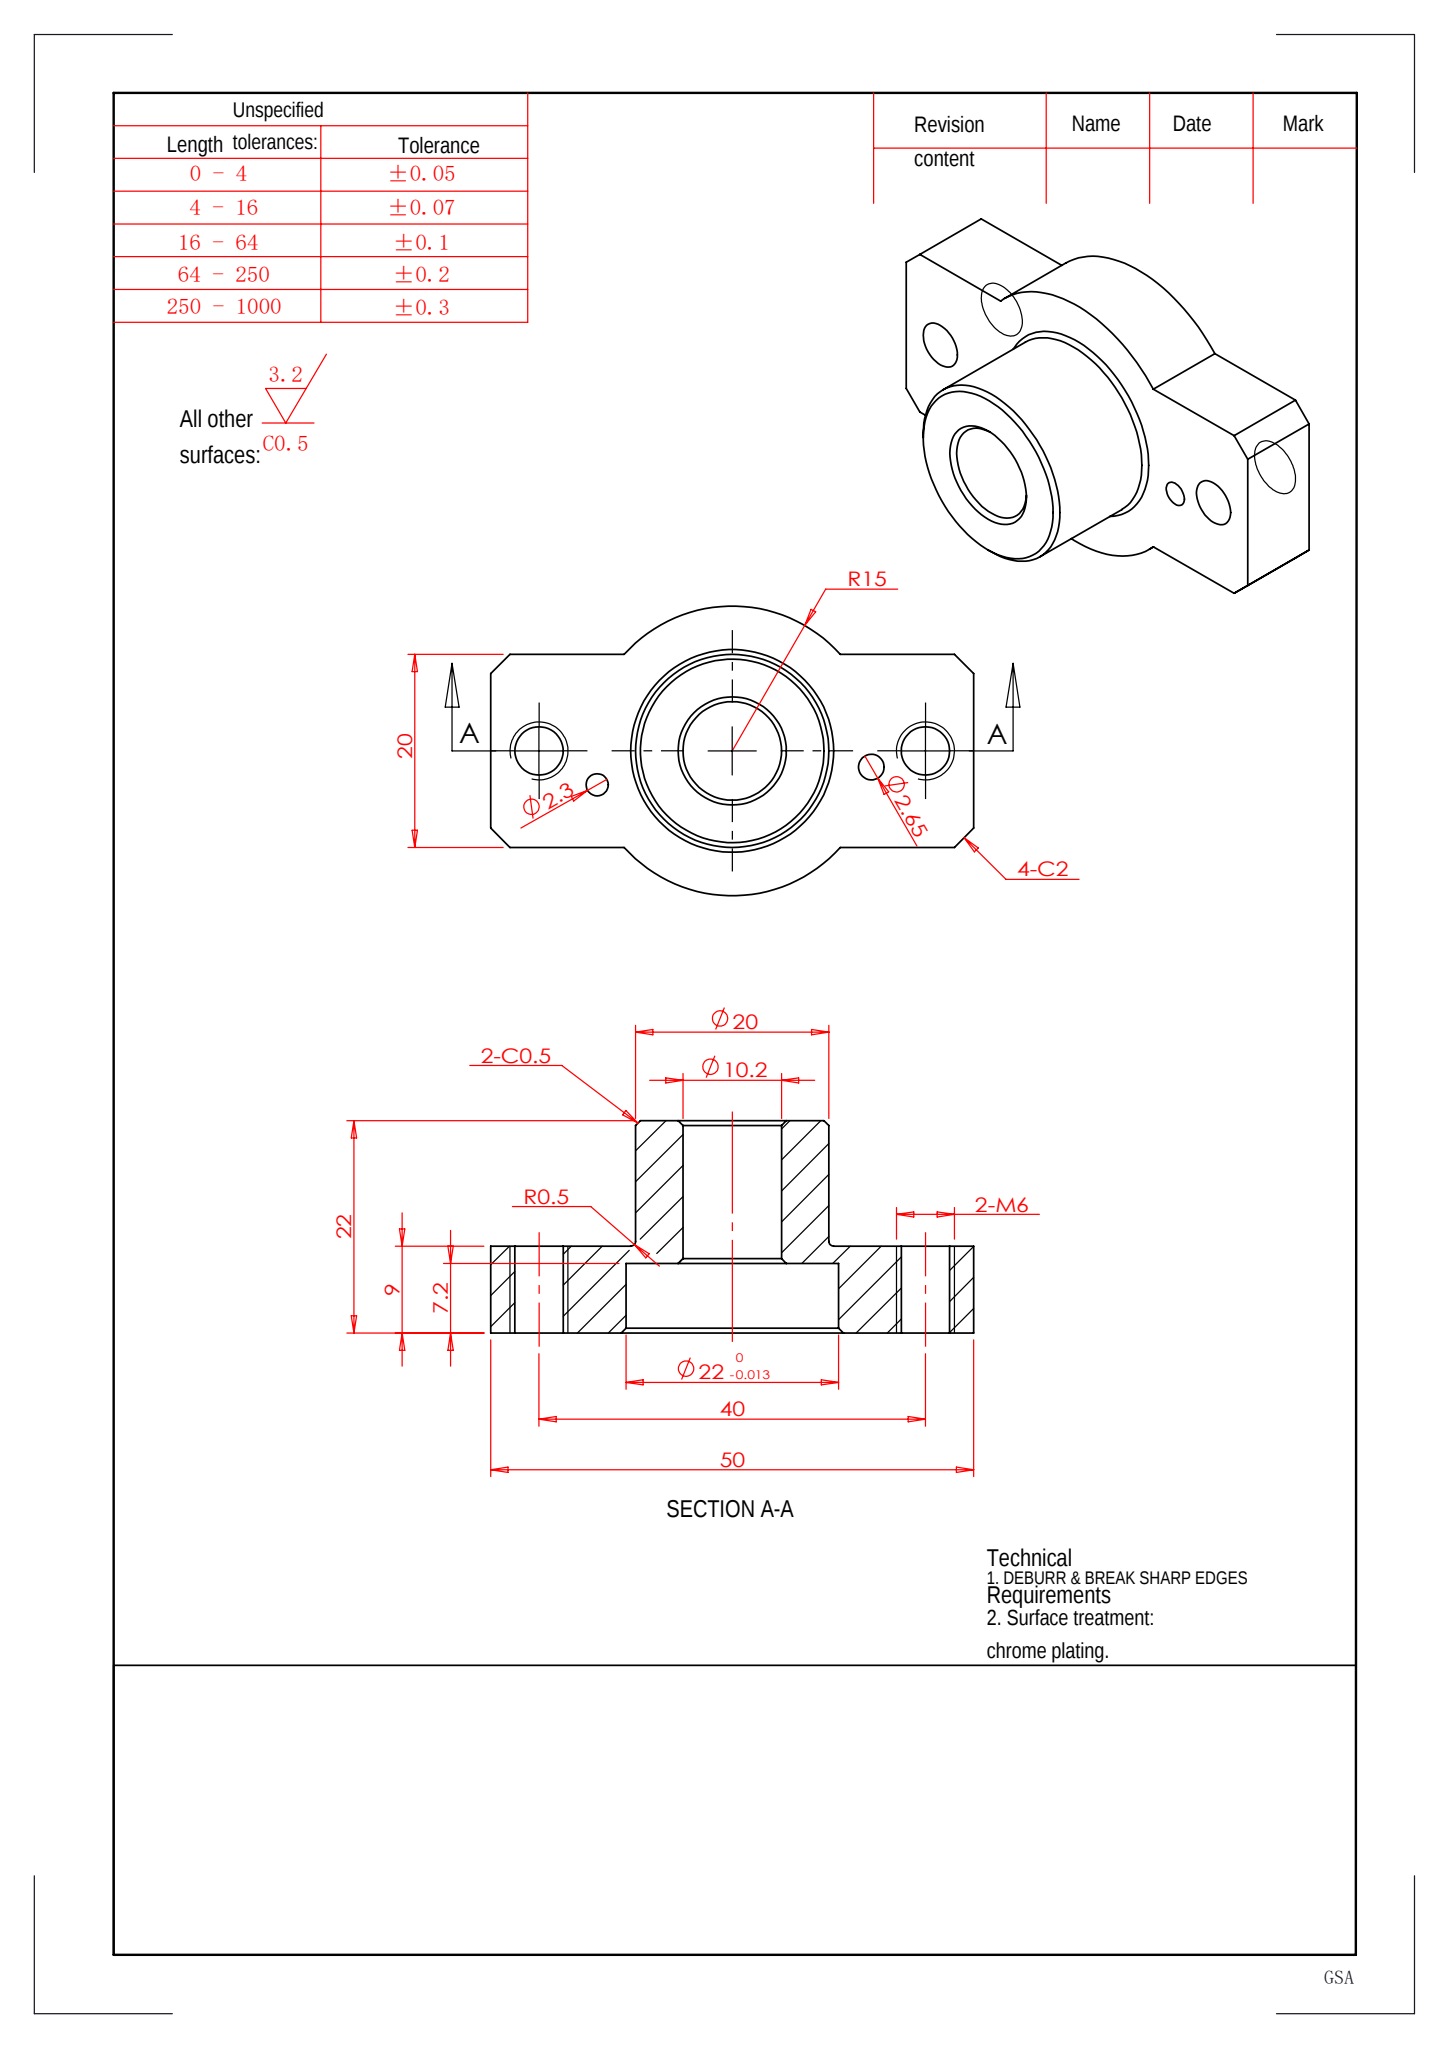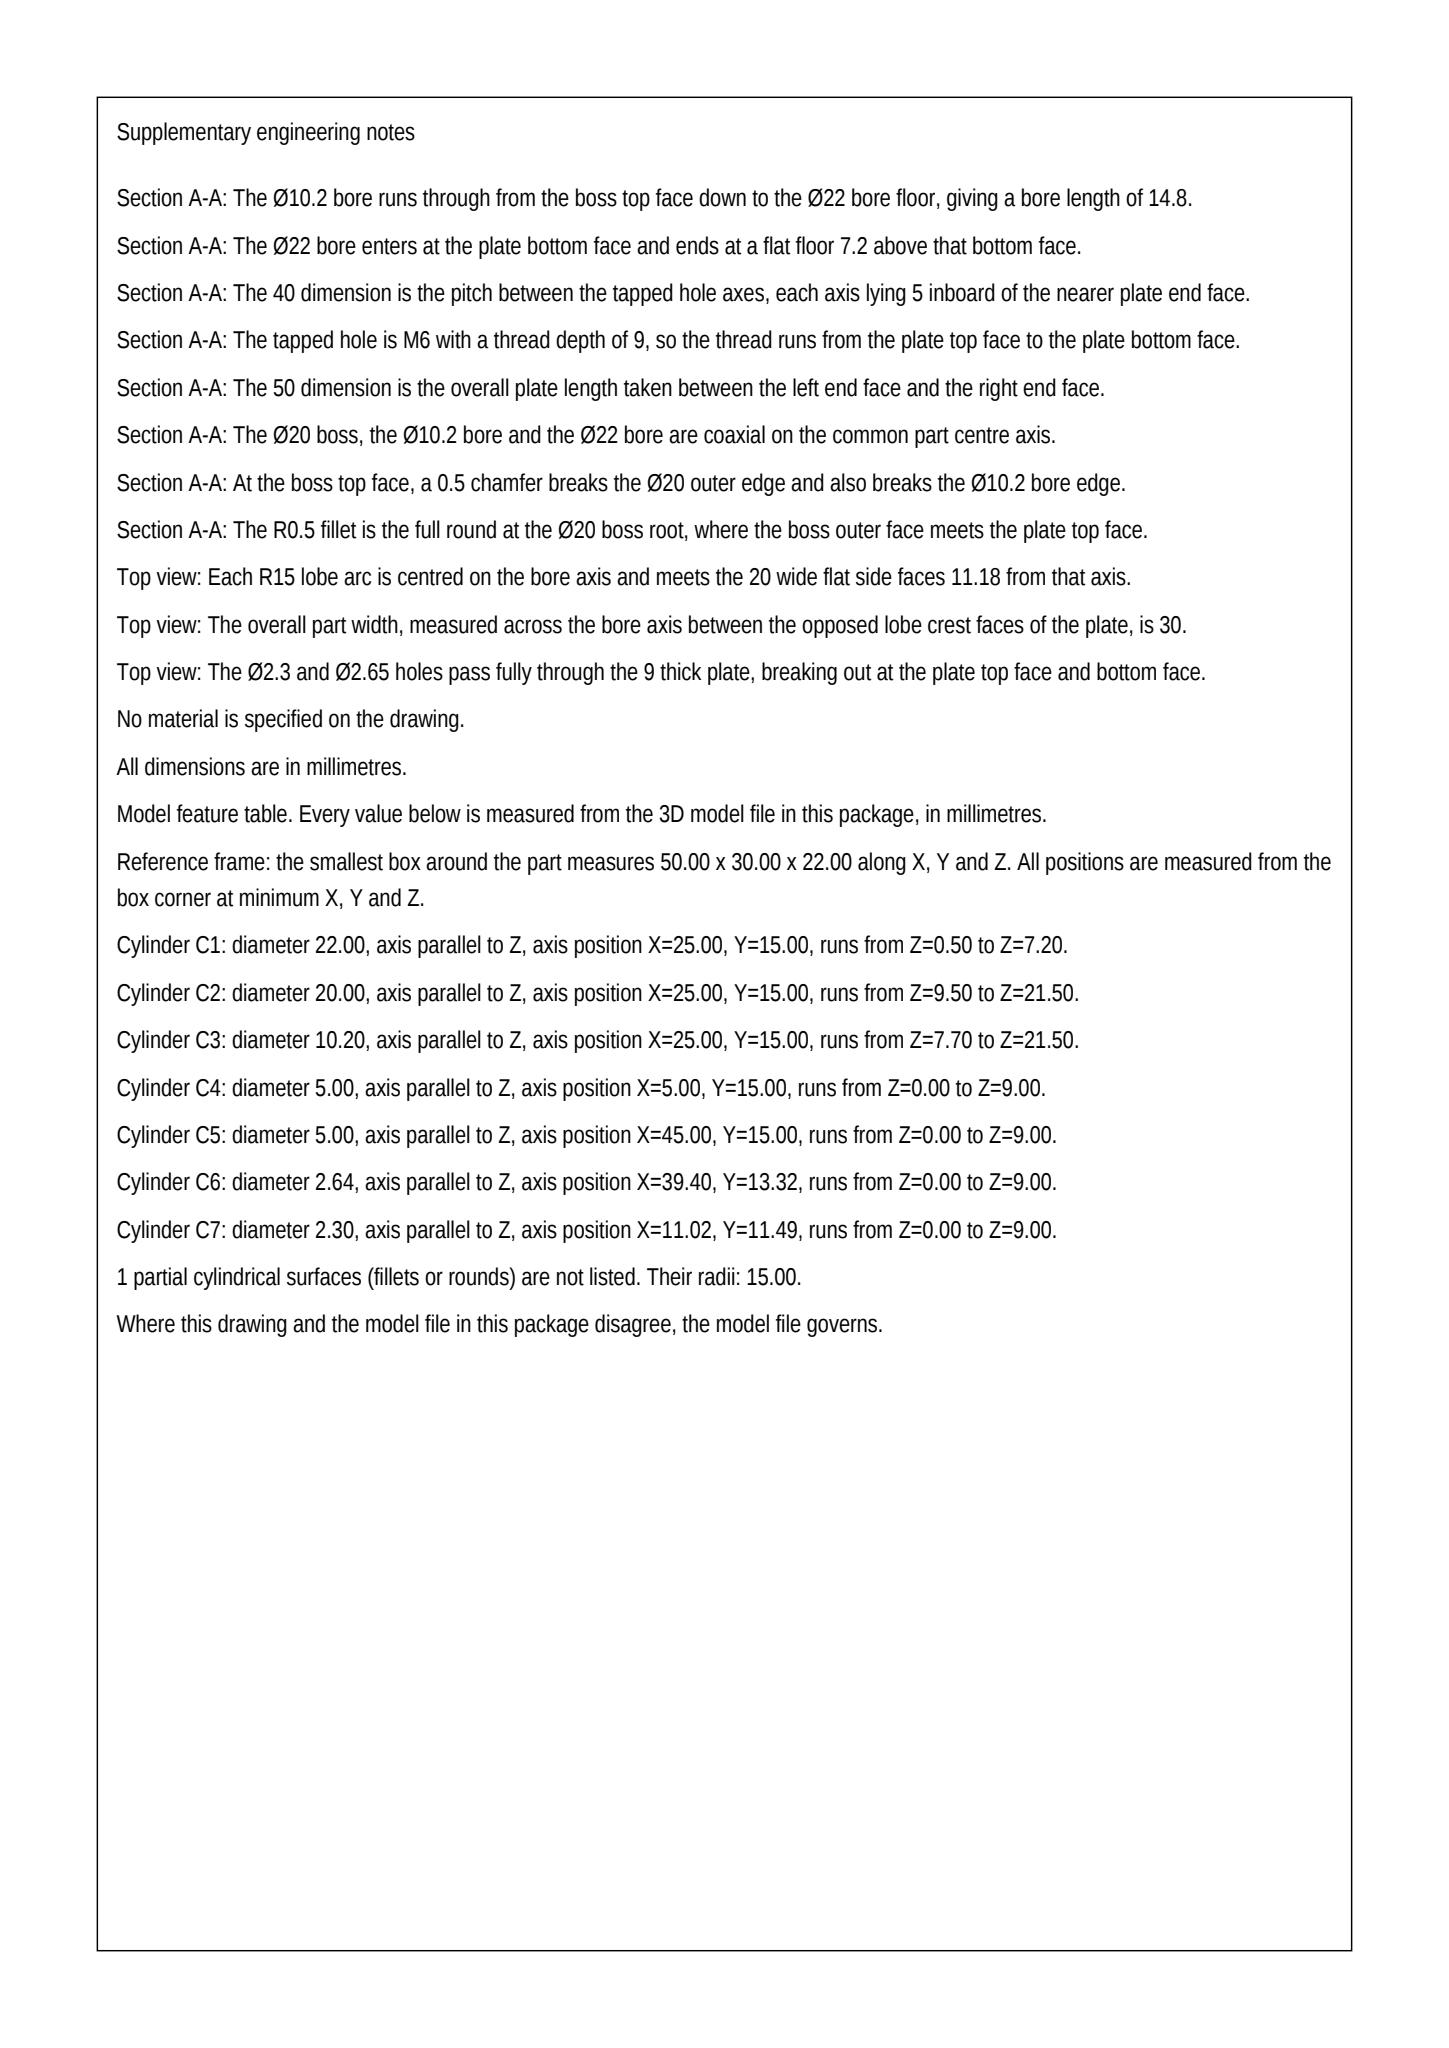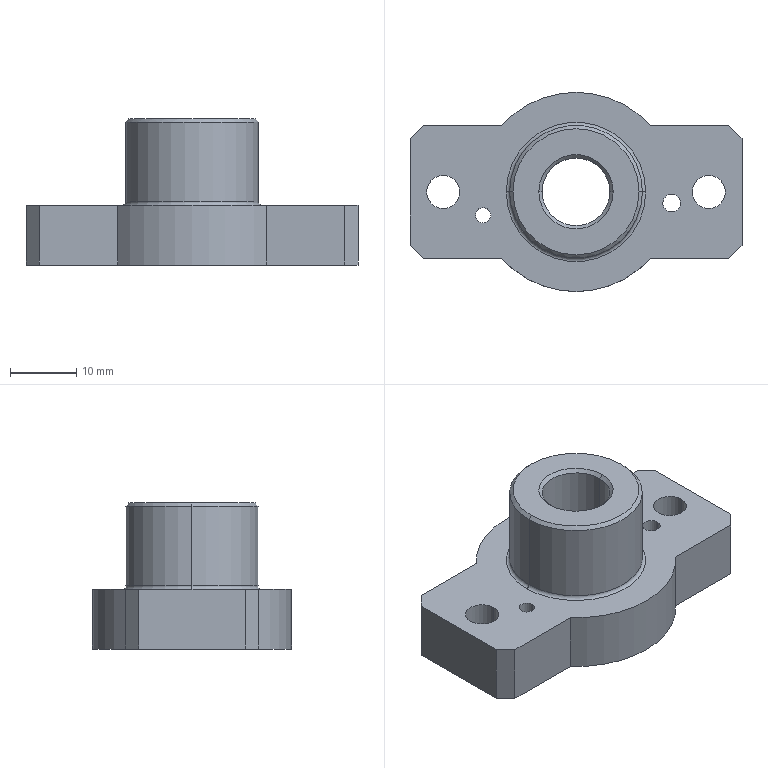Part | SolidWorks | mm | 1 solid | 40 faces | box 50 x 30 x 22 mm | volume 9998 mm3 | cylinder 16 | plane 14 | cone 8 | torus 2 | commonest cylinder face diameters 5 x4 2.65 x2 2.297 x2 22 x2 10.2 x2 20 x2 30 x2
build123d program:
from build123d import *

# Parameters (mm, degrees)
SKETCH1_R           = 1.5
BOSS_EXTRUDE1_DEPTH = 9
SKETCH2_R           = 10
SKETCH2_R_2         = 5.1
BOSS_EXTRUDE2_DEPTH = 13
SKETCH3_R           = 11
CUT_EXTRUDE1_DEPTH  = 7.2
SKETCH4_R           = 5.1
CUT_EXTRUDE2_DEPTH  = 32.922
CHAMFER1_SIZE       = 2
CHAMFER2_SIZE       = 0.5
FILLET1_R           = 0.5
M6_TAPPED_HOLE1_D   = 5
SKETCH7_R           = 1.325
SKETCH7_R_2         = 1.149
CUT_EXTRUDE3_DEPTH  = 27


with BuildPart() as part:
    # Sketch1 → Boss-Extrude1 (new body)
    with BuildSketch(Plane.XY):
        with BuildLine():
            Line((-25, -10), (-11.18, -10))
            ThreePointArc((-11.18, -10), (0, -15), (11.18, -10))
            Line((11.18, -10), (25, -10))
            Line((25, -10), (25, 10))
            Line((25, 10), (11.18, 10))
            ThreePointArc((11.18, 10), (0, 15), (-11.18, 10))
            Line((-11.18, 10), (-25, 10))
            Line((-25, 10), (-25, -10))
        make_face()
        with Locations((-20, 0)):
            Circle(SKETCH1_R, mode=Mode.SUBTRACT)
        with Locations((20, 0)):
            Circle(SKETCH1_R, mode=Mode.SUBTRACT)
    extrude(amount=BOSS_EXTRUDE1_DEPTH)

    # Sketch2 → Boss-Extrude2 (add)
    with BuildSketch(Plane.XY.offset(9)):
        with Locations(Location((0, 0, 0), (0, 0, 180))):
            Circle(SKETCH2_R)
        with Locations(Location((0, 0, 0), (0, 0, 180))):
            Circle(SKETCH2_R_2, mode=Mode.SUBTRACT)
    extrude(amount=BOSS_EXTRUDE2_DEPTH)

    # Sketch3 → Cut-Extrude1 (cut)
    with BuildSketch(Plane(origin=(0, 0, 0), x_dir=(-1, 0, 0), z_dir=(0, 0, -1))):
        Circle(SKETCH3_R)
    extrude(amount=-CUT_EXTRUDE1_DEPTH, mode=Mode.SUBTRACT)

    # Sketch4 → Cut-Extrude2 (cut, through all)
    with BuildSketch(Plane.XY.offset(9)):
        with Locations(Location((0, 0, 0), (0, 0, 180))):
            Circle(SKETCH4_R)
    extrude(amount=-CUT_EXTRUDE2_DEPTH, mode=Mode.SUBTRACT)

    # Chamfer1
    chamfer1_edges = [part.edges().sort_by_distance(p)[0] for p in [
        (25, 10, 4.5),
        (25, -10, 4.5),
        (-25, -10, 4.5),
        (-25, 10, 4.5),
    ]]
    chamfer(chamfer1_edges, length=CHAMFER1_SIZE)

    # Chamfer2
    chamfer2_edges = [part.edges().sort_by_distance(p)[0] for p in [
        (10, 0, 22),
        (5.1, 0, 22),
        (11, 0, 0),
        (5.1, 0, 7.2),
    ]]
    chamfer(chamfer2_edges, length=CHAMFER2_SIZE)

    # Fillet1
    fillet1_edges = [part.edges().sort_by_distance(p)[0] for p in [
        (10, 0, 9),
    ]]
    fillet(fillet1_edges, radius=FILLET1_R)

    # M6 Tapped Hole1 (through all)
    with Locations(Plane(origin=(20, 0, 0), x_dir=(-1, 0, 0), z_dir=(0, 0, -1))):
        with Locations((0, 0), (40, 0)):
            Hole(M6_TAPPED_HOLE1_D / 2)

    # Sketch7 → Cut-Extrude3 (cut)
    with BuildSketch(Plane(origin=(0, 0, 0), x_dir=(-1, 0, 0), z_dir=(0, 0, -1))):
        with Locations((-14.402, -1.676)):
            Circle(SKETCH7_R)
        with Locations((13.983, -3.509)):
            Circle(SKETCH7_R_2)
    extrude(amount=-CUT_EXTRUDE3_DEPTH, mode=Mode.SUBTRACT)


solid = part.part